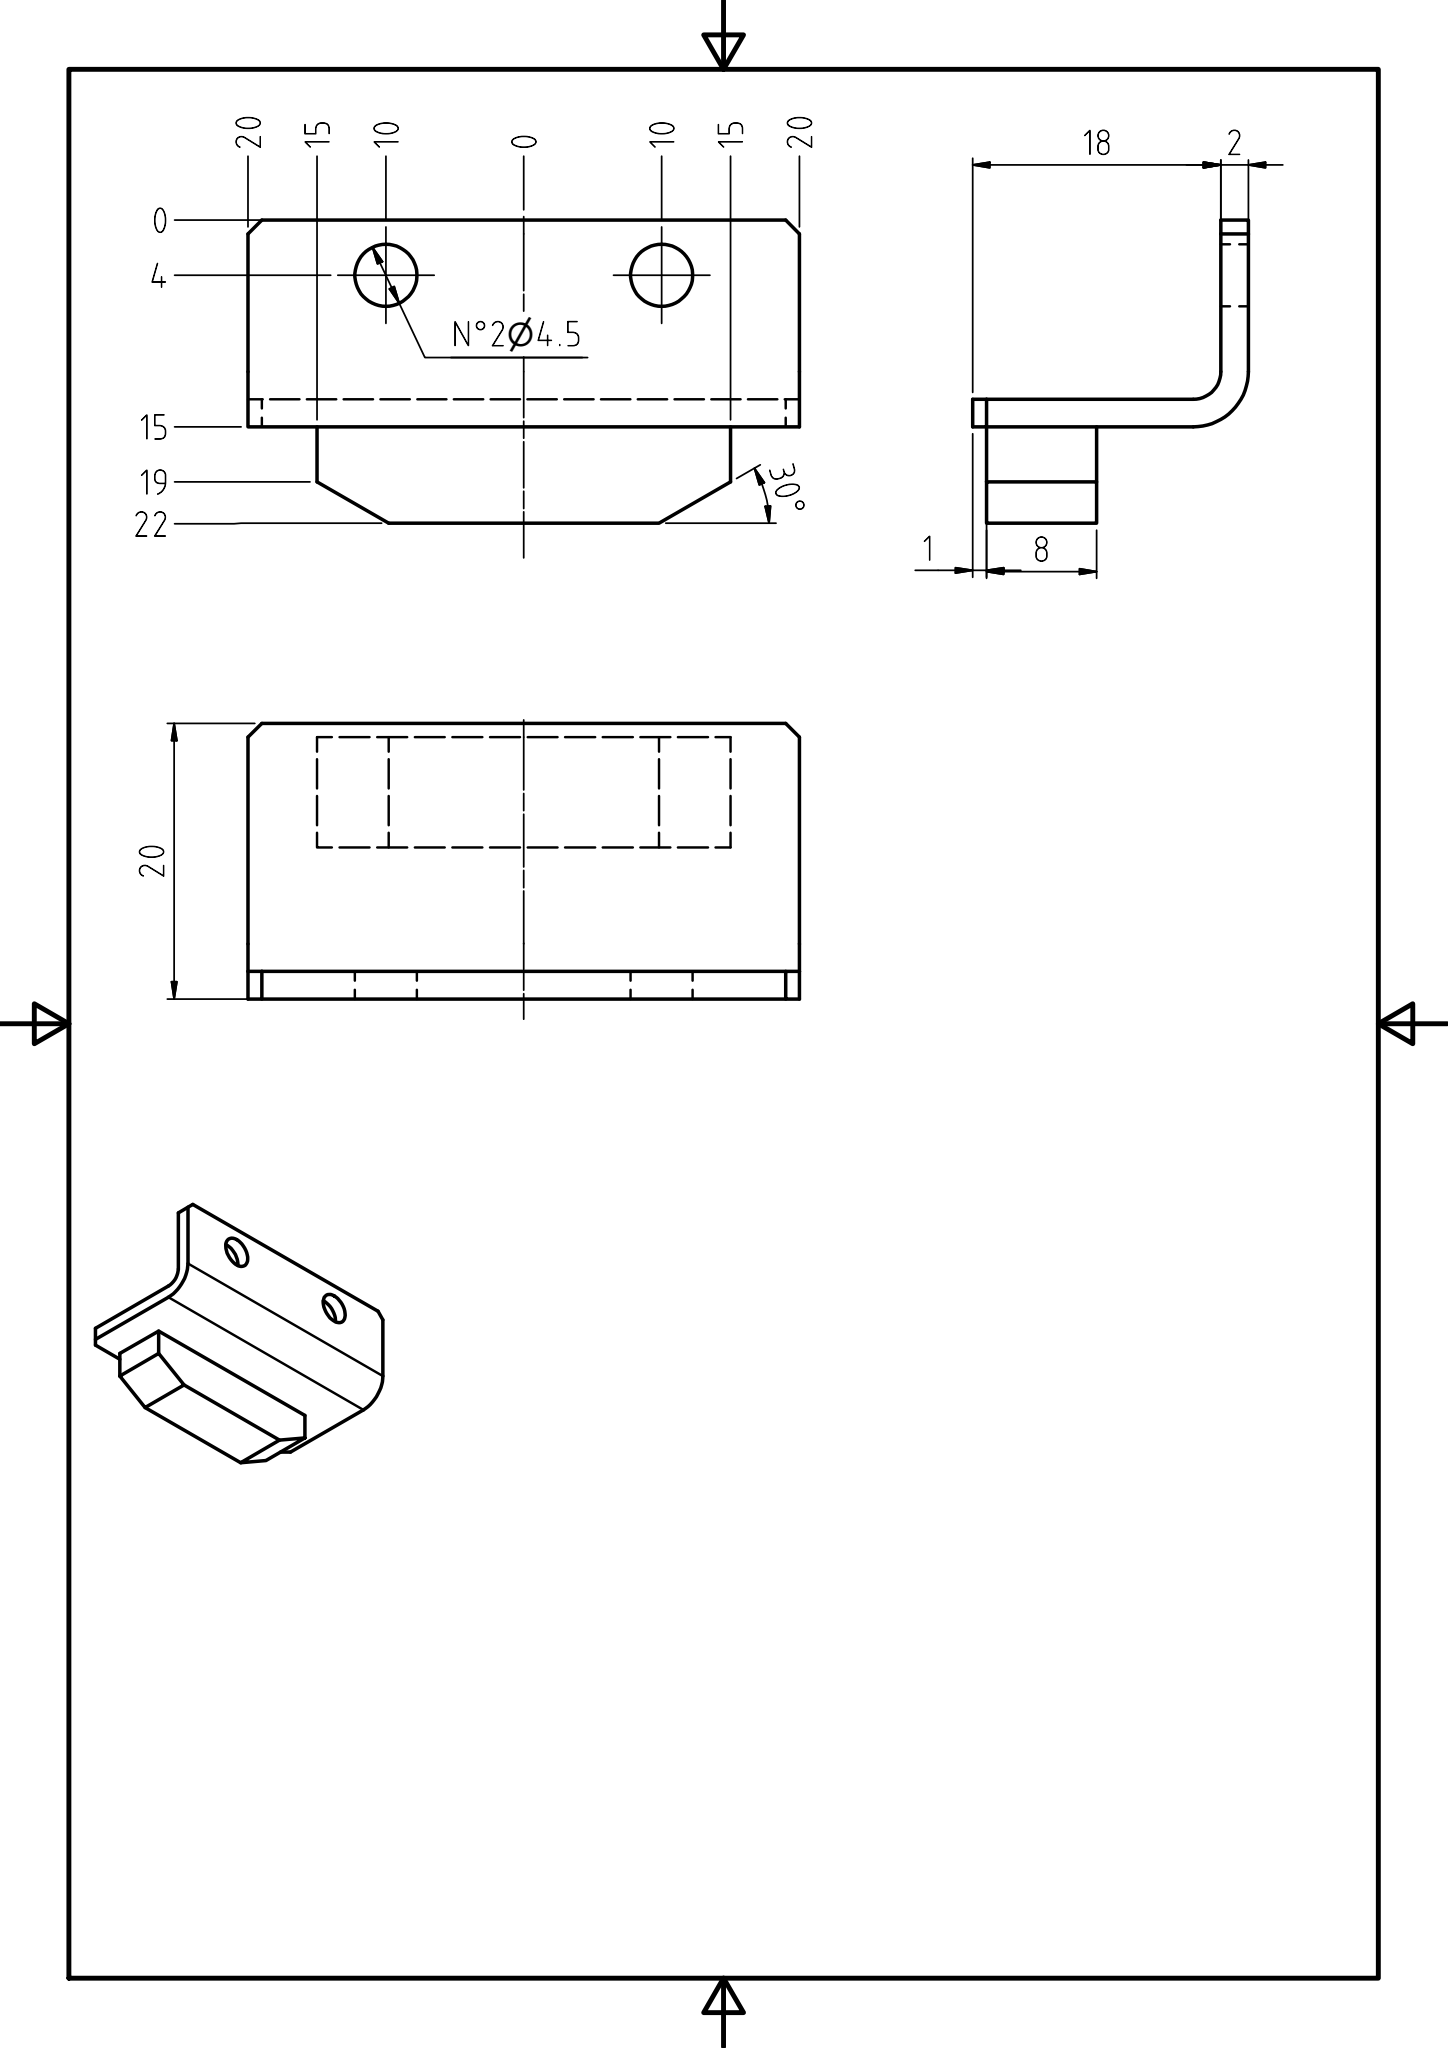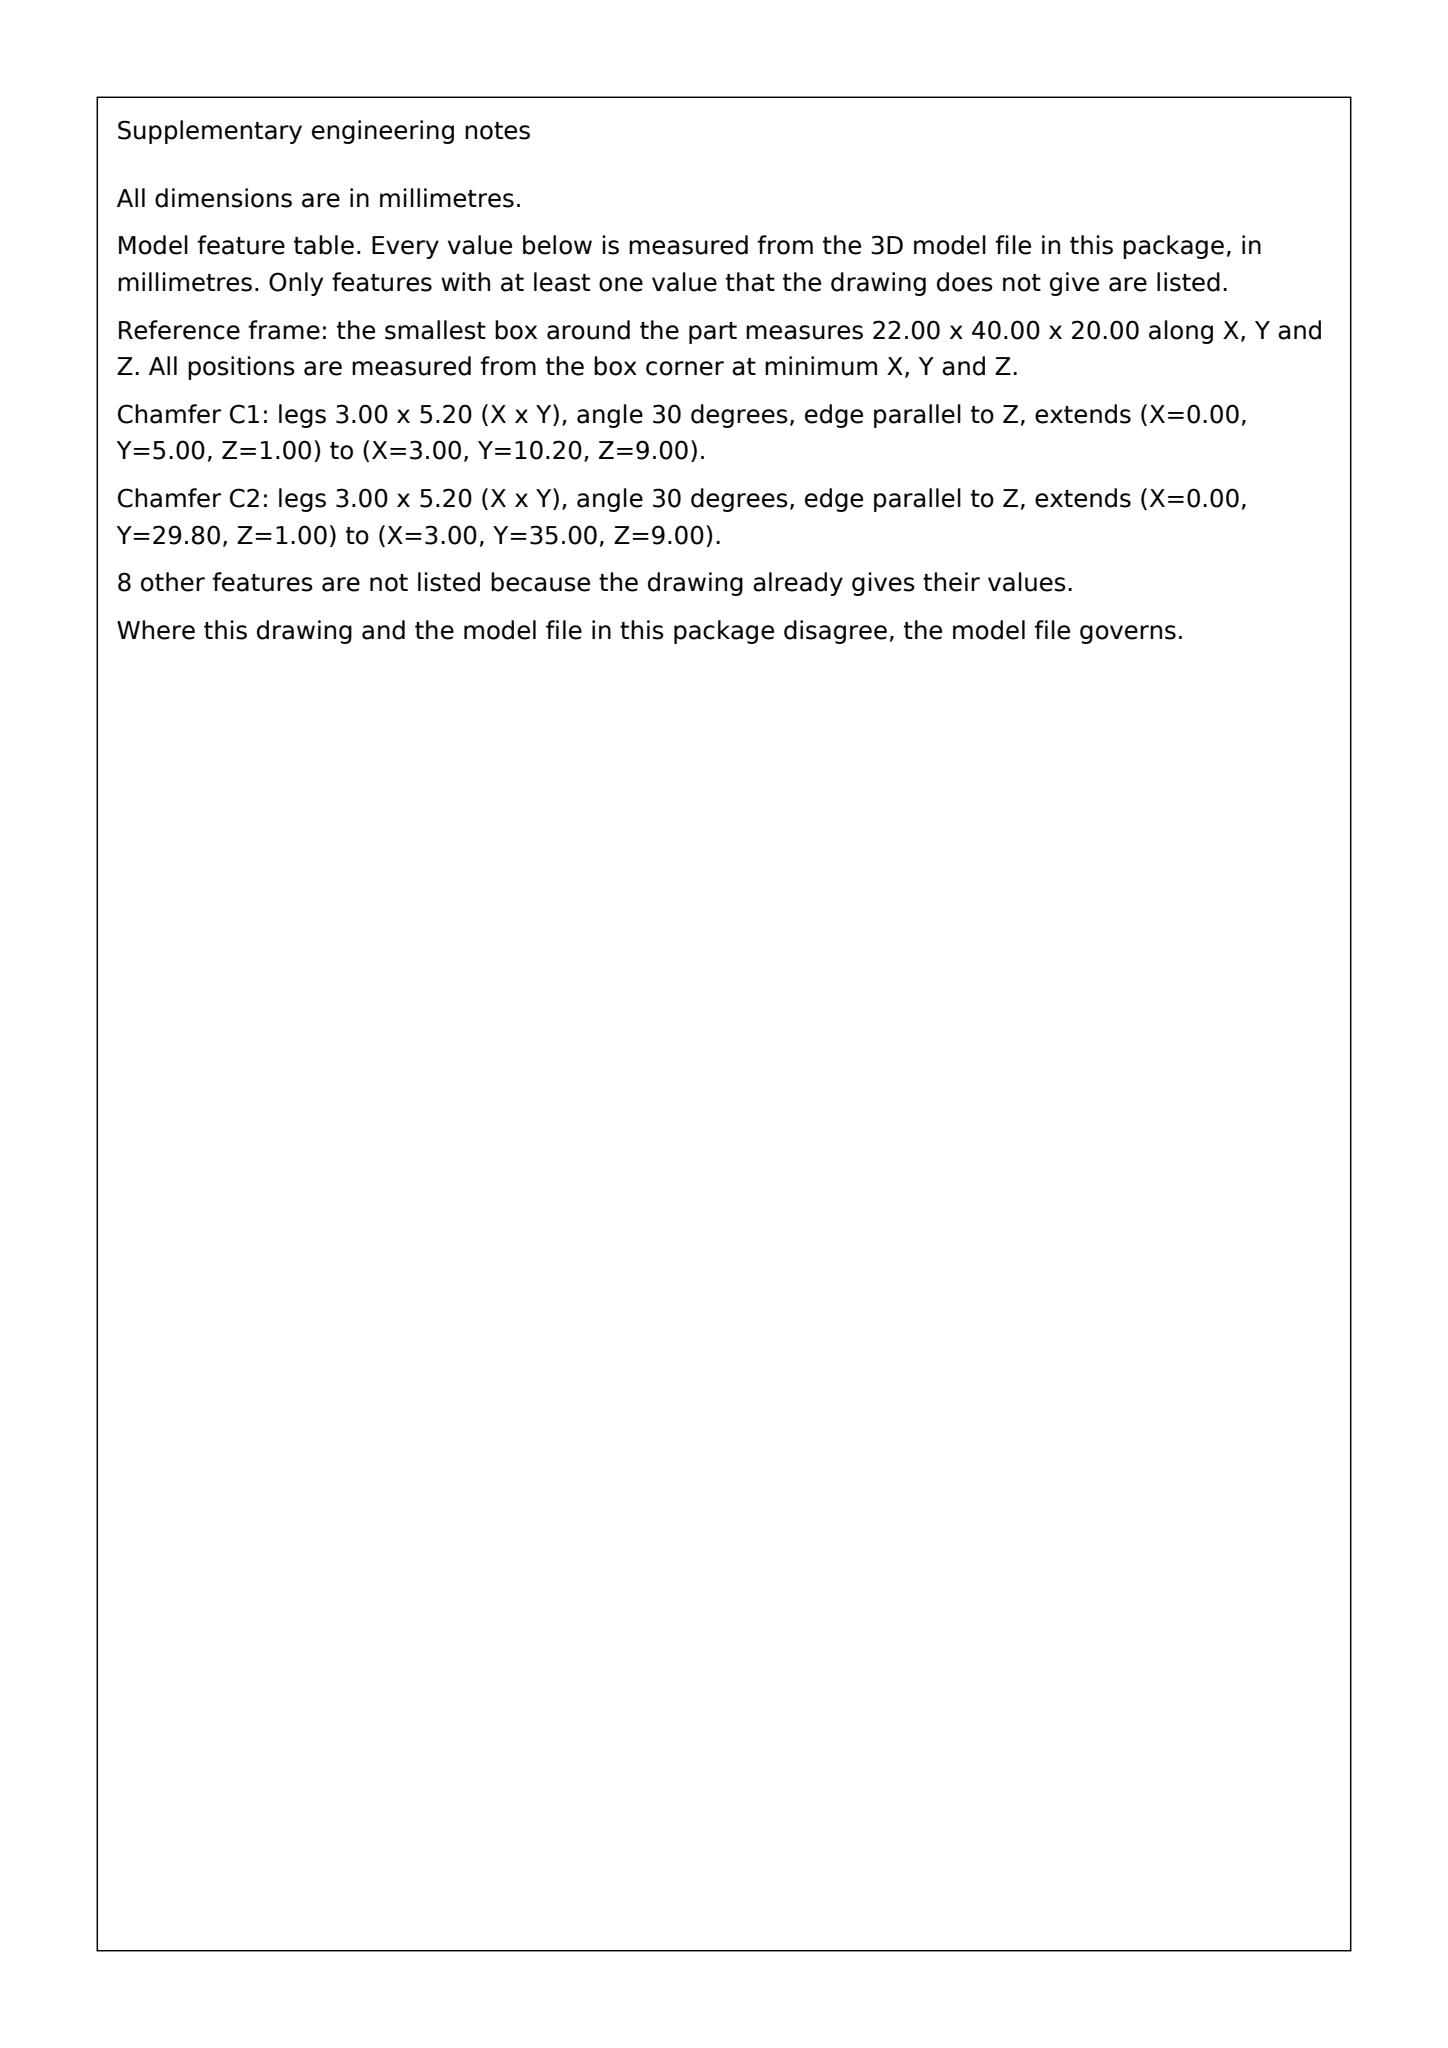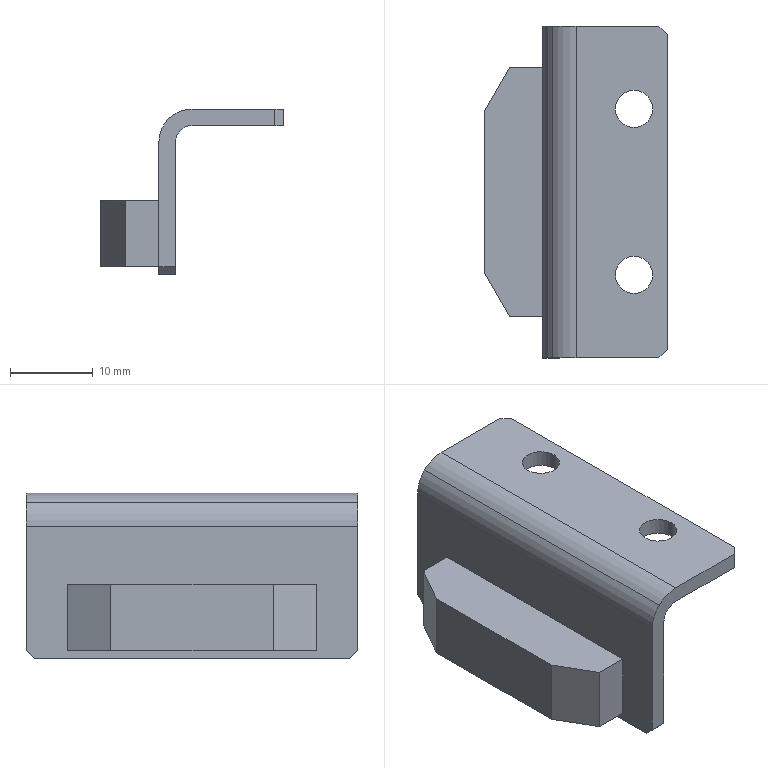Part | SolidWorks | mm | 1 solid | 27 faces | box 22 x 40 x 20 mm | volume 4025 mm3 | plane 19 | cylinder 8 | commonest cylinder face diameters 4.5 x4 4 x2 8 x2
STEP:
#1=CARTESIAN_POINT('',(-5.5,40.,6.));
#2=VERTEX_POINT('',#1);
#3=CARTESIAN_POINT('',(-4.914,40.,7.414));
#4=VERTEX_POINT('',#3);
#5=CARTESIAN_POINT('',(-3.5,40.,6.));
#6=DIRECTION('',(0.,1.,0.));
#7=DIRECTION('',(-0.7071,0.,0.7071));
#8=AXIS2_PLACEMENT_3D('',#5,#6,#7);
#9=CIRCLE('',#8,2.);
#10=EDGE_CURVE('',#2,#4,#9,.T.);
#11=ORIENTED_EDGE('',*,*,#10,.T.);
#12=CARTESIAN_POINT('',(-4.914,0.,7.414));
#13=VERTEX_POINT('',#12);
#14=CARTESIAN_POINT('',(-4.914,40.,7.414));
#15=DIRECTION('',(0.,-1.,0.));
#16=VECTOR('',#15,1000.);
#17=LINE('',#14,#16);
#18=EDGE_CURVE('',#4,#13,#17,.T.);
#19=ORIENTED_EDGE('',*,*,#18,.T.);
#20=CARTESIAN_POINT('',(-5.5,0.,6.));
#21=VERTEX_POINT('',#20);
#22=CARTESIAN_POINT('',(-3.5,0.,6.));
#23=DIRECTION('',(0.,-1.,0.));
#24=DIRECTION('',(-0.7071,0.,0.7071));
#25=AXIS2_PLACEMENT_3D('',#22,#23,#24);
#26=CIRCLE('',#25,2.);
#27=EDGE_CURVE('',#13,#21,#26,.T.);
#28=ORIENTED_EDGE('',*,*,#27,.T.);
#29=CARTESIAN_POINT('',(-5.5,40.,6.));
#30=DIRECTION('',(0.,1.,0.));
#31=VECTOR('',#30,1000.);
#32=LINE('',#29,#31);
#33=EDGE_CURVE('',#21,#2,#32,.T.);
#34=ORIENTED_EDGE('',*,*,#33,.T.);
#35=EDGE_LOOP('',(#11,#19,#28,#34));
#36=FACE_OUTER_BOUND('',#35,.T.);
#37=CARTESIAN_POINT('',(-3.5,40.,6.));
#38=DIRECTION('',(0.,-1.,0.));
#39=DIRECTION('',(-0.7071,0.,0.7071));
#40=AXIS2_PLACEMENT_3D('',#37,#38,#39);
#41=CYLINDRICAL_SURFACE('',#40,2.);
#42=ADVANCED_FACE('',(#36),#41,.F.);
#43=CARTESIAN_POINT('',(-7.5,0.,6.));
#44=VERTEX_POINT('',#43);
#45=CARTESIAN_POINT('',(-6.328,0.,8.828));
#46=VERTEX_POINT('',#45);
#47=CARTESIAN_POINT('',(-3.5,0.,6.));
#48=DIRECTION('',(0.,1.,0.));
#49=DIRECTION('',(-0.7071,0.,0.7071));
#50=AXIS2_PLACEMENT_3D('',#47,#48,#49);
#51=CIRCLE('',#50,4.);
#52=EDGE_CURVE('',#44,#46,#51,.T.);
#53=ORIENTED_EDGE('',*,*,#52,.T.);
#54=CARTESIAN_POINT('',(-6.328,40.,8.828));
#55=VERTEX_POINT('',#54);
#56=CARTESIAN_POINT('',(-6.328,0.,8.828));
#57=DIRECTION('',(0.,1.,0.));
#58=VECTOR('',#57,1000.);
#59=LINE('',#56,#58);
#60=EDGE_CURVE('',#46,#55,#59,.T.);
#61=ORIENTED_EDGE('',*,*,#60,.T.);
#62=CARTESIAN_POINT('',(-7.5,40.,6.));
#63=VERTEX_POINT('',#62);
#64=CARTESIAN_POINT('',(-3.5,40.,6.));
#65=DIRECTION('',(0.,-1.,0.));
#66=DIRECTION('',(-0.7071,0.,0.7071));
#67=AXIS2_PLACEMENT_3D('',#64,#65,#66);
#68=CIRCLE('',#67,4.);
#69=EDGE_CURVE('',#55,#63,#68,.T.);
#70=ORIENTED_EDGE('',*,*,#69,.T.);
#71=CARTESIAN_POINT('',(-7.5,0.,6.));
#72=DIRECTION('',(0.,-1.,0.));
#73=VECTOR('',#72,1000.);
#74=LINE('',#71,#73);
#75=EDGE_CURVE('',#63,#44,#74,.T.);
#76=ORIENTED_EDGE('',*,*,#75,.T.);
#77=EDGE_LOOP('',(#53,#61,#70,#76));
#78=FACE_OUTER_BOUND('',#77,.T.);
#79=CARTESIAN_POINT('',(-3.5,0.,6.));
#80=DIRECTION('',(0.,1.,0.));
#81=DIRECTION('',(-0.7071,0.,0.7071));
#82=AXIS2_PLACEMENT_3D('',#79,#80,#81);
#83=CYLINDRICAL_SURFACE('',#82,4.);
#84=ADVANCED_FACE('',(#78),#83,.T.);
#85=CARTESIAN_POINT('',(5.75,30.,10.));
#86=VERTEX_POINT('',#85);
#87=CARTESIAN_POINT('',(1.25,30.,10.));
#88=VERTEX_POINT('',#87);
#89=CARTESIAN_POINT('',(3.5,30.,10.));
#90=DIRECTION('',(-0.,0.,-1.));
#91=DIRECTION('',(-1.,0.,0.));
#92=AXIS2_PLACEMENT_3D('',#89,#90,#91);
#93=CIRCLE('',#92,2.25);
#94=EDGE_CURVE('',#86,#88,#93,.T.);
#95=ORIENTED_EDGE('',*,*,#94,.F.);
#96=CARTESIAN_POINT('',(5.75,30.,8.));
#97=VERTEX_POINT('',#96);
#98=CARTESIAN_POINT('',(5.75,30.,12.4));
#99=DIRECTION('',(-0.,0.,-1.));
#100=VECTOR('',#99,1000.);
#101=LINE('',#98,#100);
#102=EDGE_CURVE('',#86,#97,#101,.T.);
#103=ORIENTED_EDGE('',*,*,#102,.T.);
#104=CARTESIAN_POINT('',(1.25,30.,8.));
#105=VERTEX_POINT('',#104);
#106=CARTESIAN_POINT('',(3.5,30.,8.));
#107=DIRECTION('',(0.,0.,1.));
#108=DIRECTION('',(-1.,0.,0.));
#109=AXIS2_PLACEMENT_3D('',#106,#107,#108);
#110=CIRCLE('',#109,2.25);
#111=EDGE_CURVE('',#105,#97,#110,.T.);
#112=ORIENTED_EDGE('',*,*,#111,.F.);
#113=CARTESIAN_POINT('',(1.25,30.,12.4));
#114=DIRECTION('',(-0.,0.,-1.));
#115=VECTOR('',#114,1000.);
#116=LINE('',#113,#115);
#117=EDGE_CURVE('',#88,#105,#116,.T.);
#118=ORIENTED_EDGE('',*,*,#117,.F.);
#119=EDGE_LOOP('',(#95,#103,#112,#118));
#120=FACE_OUTER_BOUND('',#119,.T.);
#121=CARTESIAN_POINT('',(3.5,30.,12.4));
#122=DIRECTION('',(-0.,0.,-1.));
#123=DIRECTION('',(-1.,0.,0.));
#124=AXIS2_PLACEMENT_3D('',#121,#122,#123);
#125=CYLINDRICAL_SURFACE('',#124,2.25);
#126=ADVANCED_FACE('',(#120),#125,.F.);
#127=CARTESIAN_POINT('',(5.75,10.,10.));
#128=VERTEX_POINT('',#127);
#129=CARTESIAN_POINT('',(1.25,10.,10.));
#130=VERTEX_POINT('',#129);
#131=CARTESIAN_POINT('',(3.5,10.,10.));
#132=DIRECTION('',(-0.,0.,-1.));
#133=DIRECTION('',(-1.,0.,0.));
#134=AXIS2_PLACEMENT_3D('',#131,#132,#133);
#135=CIRCLE('',#134,2.25);
#136=EDGE_CURVE('',#128,#130,#135,.T.);
#137=ORIENTED_EDGE('',*,*,#136,.F.);
#138=CARTESIAN_POINT('',(5.75,10.,8.));
#139=VERTEX_POINT('',#138);
#140=CARTESIAN_POINT('',(5.75,10.,12.4));
#141=DIRECTION('',(-0.,0.,-1.));
#142=VECTOR('',#141,1000.);
#143=LINE('',#140,#142);
#144=EDGE_CURVE('',#128,#139,#143,.T.);
#145=ORIENTED_EDGE('',*,*,#144,.T.);
#146=CARTESIAN_POINT('',(1.25,10.,8.));
#147=VERTEX_POINT('',#146);
#148=CARTESIAN_POINT('',(3.5,10.,8.));
#149=DIRECTION('',(0.,0.,1.));
#150=DIRECTION('',(-1.,0.,0.));
#151=AXIS2_PLACEMENT_3D('',#148,#149,#150);
#152=CIRCLE('',#151,2.25);
#153=EDGE_CURVE('',#147,#139,#152,.T.);
#154=ORIENTED_EDGE('',*,*,#153,.F.);
#155=CARTESIAN_POINT('',(1.25,10.,12.4));
#156=DIRECTION('',(-0.,0.,-1.));
#157=VECTOR('',#156,1000.);
#158=LINE('',#155,#157);
#159=EDGE_CURVE('',#130,#147,#158,.T.);
#160=ORIENTED_EDGE('',*,*,#159,.F.);
#161=EDGE_LOOP('',(#137,#145,#154,#160));
#162=FACE_OUTER_BOUND('',#161,.T.);
#163=CARTESIAN_POINT('',(3.5,10.,12.4));
#164=DIRECTION('',(-0.,0.,-1.));
#165=DIRECTION('',(-1.,0.,0.));
#166=AXIS2_PLACEMENT_3D('',#163,#164,#165);
#167=CYLINDRICAL_SURFACE('',#166,2.25);
#168=ADVANCED_FACE('',(#162),#167,.F.);
#169=CARTESIAN_POINT('',(-7.5,0.,-9.));
#170=VERTEX_POINT('',#169);
#171=CARTESIAN_POINT('',(-7.5,1.,-10.));
#172=VERTEX_POINT('',#171);
#173=CARTESIAN_POINT('',(-7.5,0.5,-9.5));
#174=DIRECTION('',(0.,0.7071,-0.7071));
#175=VECTOR('',#174,1000.);
#176=LINE('',#173,#175);
#177=EDGE_CURVE('',#170,#172,#176,.T.);
#178=ORIENTED_EDGE('',*,*,#177,.T.);
#179=CARTESIAN_POINT('',(-5.5,1.,-10.));
#180=VERTEX_POINT('',#179);
#181=CARTESIAN_POINT('',(3.75,1.,-10.));
#182=DIRECTION('',(1.,0.,0.));
#183=VECTOR('',#182,1000.);
#184=LINE('',#181,#183);
#185=EDGE_CURVE('',#172,#180,#184,.T.);
#186=ORIENTED_EDGE('',*,*,#185,.T.);
#187=CARTESIAN_POINT('',(-5.5,0.,-9.));
#188=VERTEX_POINT('',#187);
#189=CARTESIAN_POINT('',(-5.5,6.,-15.));
#190=DIRECTION('',(0.,-0.7071,0.7071));
#191=VECTOR('',#190,1000.);
#192=LINE('',#189,#191);
#193=EDGE_CURVE('',#180,#188,#192,.T.);
#194=ORIENTED_EDGE('',*,*,#193,.T.);
#195=CARTESIAN_POINT('',(3.75,0.,-9.));
#196=DIRECTION('',(-1.,0.,-0.));
#197=VECTOR('',#196,1000.);
#198=LINE('',#195,#197);
#199=EDGE_CURVE('',#188,#170,#198,.T.);
#200=ORIENTED_EDGE('',*,*,#199,.T.);
#201=EDGE_LOOP('',(#178,#186,#194,#200));
#202=FACE_OUTER_BOUND('',#201,.T.);
#203=CARTESIAN_POINT('',(3.75,0.5,-9.5));
#204=DIRECTION('',(0.,-0.7071,-0.7071));
#205=DIRECTION('',(0.,-0.7071,0.7071));
#206=AXIS2_PLACEMENT_3D('',#203,#204,#205);
#207=PLANE('',#206);
#208=ADVANCED_FACE('',(#202),#207,.T.);
#209=ORIENTED_EDGE('',*,*,#199,.F.);
#210=CARTESIAN_POINT('',(-5.5,0.,4.));
#211=DIRECTION('',(0.,0.,1.));
#212=VECTOR('',#211,1000.);
#213=LINE('',#210,#212);
#214=EDGE_CURVE('',#188,#21,#213,.T.);
#215=ORIENTED_EDGE('',*,*,#214,.T.);
#216=ORIENTED_EDGE('',*,*,#27,.F.);
#217=CARTESIAN_POINT('',(-3.5,0.,8.));
#218=VERTEX_POINT('',#217);
#219=CARTESIAN_POINT('',(-3.5,0.,6.));
#220=DIRECTION('',(0.,-1.,0.));
#221=DIRECTION('',(-0.7071,0.,0.7071));
#222=AXIS2_PLACEMENT_3D('',#219,#220,#221);
#223=CIRCLE('',#222,2.);
#224=EDGE_CURVE('',#218,#13,#223,.T.);
#225=ORIENTED_EDGE('',*,*,#224,.F.);
#226=CARTESIAN_POINT('',(6.5,0.,8.));
#227=VERTEX_POINT('',#226);
#228=CARTESIAN_POINT('',(7.237,0.,8.));
#229=DIRECTION('',(1.,0.,-0.));
#230=VECTOR('',#229,1000.);
#231=LINE('',#228,#230);
#232=EDGE_CURVE('',#218,#227,#231,.T.);
#233=ORIENTED_EDGE('',*,*,#232,.T.);
#234=CARTESIAN_POINT('',(6.5,0.,10.));
#235=VERTEX_POINT('',#234);
#236=CARTESIAN_POINT('',(6.5,0.,5.));
#237=DIRECTION('',(0.,0.,-1.));
#238=VECTOR('',#237,1000.);
#239=LINE('',#236,#238);
#240=EDGE_CURVE('',#235,#227,#239,.T.);
#241=ORIENTED_EDGE('',*,*,#240,.F.);
#242=CARTESIAN_POINT('',(-3.5,0.,10.));
#243=VERTEX_POINT('',#242);
#244=CARTESIAN_POINT('',(-7.5,0.,10.));
#245=DIRECTION('',(1.,0.,-0.));
#246=VECTOR('',#245,1000.);
#247=LINE('',#244,#246);
#248=EDGE_CURVE('',#243,#235,#247,.T.);
#249=ORIENTED_EDGE('',*,*,#248,.F.);
#250=CARTESIAN_POINT('',(-3.5,0.,6.));
#251=DIRECTION('',(0.,1.,0.));
#252=DIRECTION('',(-0.7071,0.,0.7071));
#253=AXIS2_PLACEMENT_3D('',#250,#251,#252);
#254=CIRCLE('',#253,4.);
#255=EDGE_CURVE('',#46,#243,#254,.T.);
#256=ORIENTED_EDGE('',*,*,#255,.F.);
#257=ORIENTED_EDGE('',*,*,#52,.F.);
#258=CARTESIAN_POINT('',(-7.5,0.,-10.));
#259=DIRECTION('',(0.,0.,1.));
#260=VECTOR('',#259,1000.);
#261=LINE('',#258,#260);
#262=EDGE_CURVE('',#170,#44,#261,.T.);
#263=ORIENTED_EDGE('',*,*,#262,.F.);
#264=EDGE_LOOP('',(#209,#215,#216,#225,#233,#241,#249,#256,#257,#263));
#265=FACE_OUTER_BOUND('',#264,.T.);
#266=CARTESIAN_POINT('',(0.,0.,0.));
#267=DIRECTION('',(0.,1.,0.));
#268=DIRECTION('',(1.,0.,0.));
#269=AXIS2_PLACEMENT_3D('',#266,#267,#268);
#270=PLANE('',#269);
#271=ADVANCED_FACE('',(#265),#270,.F.);
#272=ORIENTED_EDGE('',*,*,#193,.F.);
#273=CARTESIAN_POINT('',(-5.5,39.,-10.));
#274=VERTEX_POINT('',#273);
#275=CARTESIAN_POINT('',(-5.5,20.,-10.));
#276=DIRECTION('',(0.,-1.,0.));
#277=VECTOR('',#276,1000.);
#278=LINE('',#275,#277);
#279=EDGE_CURVE('',#274,#180,#278,.T.);
#280=ORIENTED_EDGE('',*,*,#279,.F.);
#281=CARTESIAN_POINT('',(-5.5,40.,-9.));
#282=VERTEX_POINT('',#281);
#283=CARTESIAN_POINT('',(-5.5,44.,-5.));
#284=DIRECTION('',(-0.,-0.7071,-0.7071));
#285=VECTOR('',#284,1000.);
#286=LINE('',#283,#285);
#287=EDGE_CURVE('',#282,#274,#286,.T.);
#288=ORIENTED_EDGE('',*,*,#287,.F.);
#289=CARTESIAN_POINT('',(-5.5,40.,4.));
#290=DIRECTION('',(-0.,0.,-1.));
#291=VECTOR('',#290,1000.);
#292=LINE('',#289,#291);
#293=EDGE_CURVE('',#2,#282,#292,.T.);
#294=ORIENTED_EDGE('',*,*,#293,.F.);
#295=ORIENTED_EDGE('',*,*,#33,.F.);
#296=ORIENTED_EDGE('',*,*,#214,.F.);
#297=EDGE_LOOP('',(#272,#280,#288,#294,#295,#296));
#298=FACE_OUTER_BOUND('',#297,.T.);
#299=CARTESIAN_POINT('',(-5.5,40.,8.));
#300=DIRECTION('',(-1.,0.,0.));
#301=DIRECTION('',(0.,1.,0.));
#302=AXIS2_PLACEMENT_3D('',#299,#300,#301);
#303=PLANE('',#302);
#304=ADVANCED_FACE('',(#298),#303,.F.);
#305=CARTESIAN_POINT('',(-7.5,39.,-10.));
#306=VERTEX_POINT('',#305);
#307=CARTESIAN_POINT('',(-7.5,40.,-9.));
#308=VERTEX_POINT('',#307);
#309=CARTESIAN_POINT('',(-7.5,29.5,-19.5));
#310=DIRECTION('',(0.,0.7071,0.7071));
#311=VECTOR('',#310,1000.);
#312=LINE('',#309,#311);
#313=EDGE_CURVE('',#306,#308,#312,.T.);
#314=ORIENTED_EDGE('',*,*,#313,.T.);
#315=CARTESIAN_POINT('',(3.75,40.,-9.));
#316=DIRECTION('',(1.,0.,0.));
#317=VECTOR('',#316,1000.);
#318=LINE('',#315,#317);
#319=EDGE_CURVE('',#308,#282,#318,.T.);
#320=ORIENTED_EDGE('',*,*,#319,.T.);
#321=ORIENTED_EDGE('',*,*,#287,.T.);
#322=CARTESIAN_POINT('',(3.75,39.,-10.));
#323=DIRECTION('',(-1.,0.,-0.));
#324=VECTOR('',#323,1000.);
#325=LINE('',#322,#324);
#326=EDGE_CURVE('',#274,#306,#325,.T.);
#327=ORIENTED_EDGE('',*,*,#326,.T.);
#328=EDGE_LOOP('',(#314,#320,#321,#327));
#329=FACE_OUTER_BOUND('',#328,.T.);
#330=CARTESIAN_POINT('',(3.75,39.5,-9.5));
#331=DIRECTION('',(0.,0.7071,-0.7071));
#332=DIRECTION('',(-1.,0.,-0.));
#333=AXIS2_PLACEMENT_3D('',#330,#331,#332);
#334=PLANE('',#333);
#335=ADVANCED_FACE('',(#329),#334,.T.);
#336=ORIENTED_EDGE('',*,*,#319,.F.);
#337=CARTESIAN_POINT('',(-7.5,40.,-10.));
#338=DIRECTION('',(0.,0.,1.));
#339=VECTOR('',#338,1000.);
#340=LINE('',#337,#339);
#341=EDGE_CURVE('',#308,#63,#340,.T.);
#342=ORIENTED_EDGE('',*,*,#341,.T.);
#343=ORIENTED_EDGE('',*,*,#69,.F.);
#344=CARTESIAN_POINT('',(-3.5,40.,10.));
#345=VERTEX_POINT('',#344);
#346=CARTESIAN_POINT('',(-3.5,40.,6.));
#347=DIRECTION('',(0.,-1.,0.));
#348=DIRECTION('',(-0.7071,0.,0.7071));
#349=AXIS2_PLACEMENT_3D('',#346,#347,#348);
#350=CIRCLE('',#349,4.);
#351=EDGE_CURVE('',#345,#55,#350,.T.);
#352=ORIENTED_EDGE('',*,*,#351,.F.);
#353=CARTESIAN_POINT('',(6.5,40.,10.));
#354=VERTEX_POINT('',#353);
#355=CARTESIAN_POINT('',(-7.5,40.,10.));
#356=DIRECTION('',(1.,0.,-0.));
#357=VECTOR('',#356,1000.);
#358=LINE('',#355,#357);
#359=EDGE_CURVE('',#345,#354,#358,.T.);
#360=ORIENTED_EDGE('',*,*,#359,.T.);
#361=CARTESIAN_POINT('',(6.5,40.,8.));
#362=VERTEX_POINT('',#361);
#363=CARTESIAN_POINT('',(6.5,40.,5.));
#364=DIRECTION('',(0.,0.,1.));
#365=VECTOR('',#364,1000.);
#366=LINE('',#363,#365);
#367=EDGE_CURVE('',#362,#354,#366,.T.);
#368=ORIENTED_EDGE('',*,*,#367,.F.);
#369=CARTESIAN_POINT('',(-3.5,40.,8.));
#370=VERTEX_POINT('',#369);
#371=CARTESIAN_POINT('',(7.237,40.,8.));
#372=DIRECTION('',(-1.,0.,0.));
#373=VECTOR('',#372,1000.);
#374=LINE('',#371,#373);
#375=EDGE_CURVE('',#362,#370,#374,.T.);
#376=ORIENTED_EDGE('',*,*,#375,.T.);
#377=CARTESIAN_POINT('',(-3.5,40.,6.));
#378=DIRECTION('',(0.,1.,0.));
#379=DIRECTION('',(-0.7071,0.,0.7071));
#380=AXIS2_PLACEMENT_3D('',#377,#378,#379);
#381=CIRCLE('',#380,2.);
#382=EDGE_CURVE('',#4,#370,#381,.T.);
#383=ORIENTED_EDGE('',*,*,#382,.F.);
#384=ORIENTED_EDGE('',*,*,#10,.F.);
#385=ORIENTED_EDGE('',*,*,#293,.T.);
#386=EDGE_LOOP('',(#336,#342,#343,#352,#360,#368,#376,#383,#384,#385));
#387=FACE_OUTER_BOUND('',#386,.T.);
#388=CARTESIAN_POINT('',(0.,40.,0.));
#389=DIRECTION('',(0.,1.,0.));
#390=DIRECTION('',(1.,0.,0.));
#391=AXIS2_PLACEMENT_3D('',#388,#389,#390);
#392=PLANE('',#391);
#393=ADVANCED_FACE('',(#387),#392,.T.);
#394=CARTESIAN_POINT('',(7.5,39.,8.));
#395=VERTEX_POINT('',#394);
#396=CARTESIAN_POINT('',(8.744,37.756,8.));
#397=DIRECTION('',(-0.7071,0.7071,0.));
#398=VECTOR('',#397,1000.);
#399=LINE('',#396,#398);
#400=EDGE_CURVE('',#395,#362,#399,.T.);
#401=ORIENTED_EDGE('',*,*,#400,.T.);
#402=ORIENTED_EDGE('',*,*,#367,.T.);
#403=CARTESIAN_POINT('',(7.5,39.,10.));
#404=VERTEX_POINT('',#403);
#405=CARTESIAN_POINT('',(13.25,33.25,10.));
#406=DIRECTION('',(0.7071,-0.7071,-0.));
#407=VECTOR('',#406,1000.);
#408=LINE('',#405,#407);
#409=EDGE_CURVE('',#354,#404,#408,.T.);
#410=ORIENTED_EDGE('',*,*,#409,.T.);
#411=CARTESIAN_POINT('',(7.5,39.,5.));
#412=DIRECTION('',(0.,0.,-1.));
#413=VECTOR('',#412,1000.);
#414=LINE('',#411,#413);
#415=EDGE_CURVE('',#404,#395,#414,.T.);
#416=ORIENTED_EDGE('',*,*,#415,.T.);
#417=EDGE_LOOP('',(#401,#402,#410,#416));
#418=FACE_OUTER_BOUND('',#417,.T.);
#419=CARTESIAN_POINT('',(7.,39.5,5.));
#420=DIRECTION('',(0.7071,0.7071,0.));
#421=DIRECTION('',(0.,0.,-1.));
#422=AXIS2_PLACEMENT_3D('',#419,#420,#421);
#423=PLANE('',#422);
#424=ADVANCED_FACE('',(#418),#423,.T.);
#425=ORIENTED_EDGE('',*,*,#400,.F.);
#426=CARTESIAN_POINT('',(7.5,1.,8.));
#427=VERTEX_POINT('',#426);
#428=CARTESIAN_POINT('',(7.5,20.,8.));
#429=DIRECTION('',(0.,1.,0.));
#430=VECTOR('',#429,1000.);
#431=LINE('',#428,#430);
#432=EDGE_CURVE('',#427,#395,#431,.T.);
#433=ORIENTED_EDGE('',*,*,#432,.F.);
#434=CARTESIAN_POINT('',(18.744,12.244,8.));
#435=DIRECTION('',(0.7071,0.7071,-0.));
#436=VECTOR('',#435,1000.);
#437=LINE('',#434,#436);
#438=EDGE_CURVE('',#227,#427,#437,.T.);
#439=ORIENTED_EDGE('',*,*,#438,.F.);
#440=ORIENTED_EDGE('',*,*,#232,.F.);
#441=CARTESIAN_POINT('',(-3.5,40.,8.));
#442=DIRECTION('',(0.,-1.,0.));
#443=VECTOR('',#442,1000.);
#444=LINE('',#441,#443);
#445=EDGE_CURVE('',#370,#218,#444,.T.);
#446=ORIENTED_EDGE('',*,*,#445,.F.);
#447=ORIENTED_EDGE('',*,*,#375,.F.);
#448=EDGE_LOOP('',(#425,#433,#439,#440,#446,#447));
#449=FACE_OUTER_BOUND('',#448,.T.);
#450=ORIENTED_EDGE('',*,*,#111,.T.);
#451=CARTESIAN_POINT('',(3.5,30.,8.));
#452=DIRECTION('',(0.,0.,1.));
#453=DIRECTION('',(-1.,0.,0.));
#454=AXIS2_PLACEMENT_3D('',#451,#452,#453);
#455=CIRCLE('',#454,2.25);
#456=EDGE_CURVE('',#97,#105,#455,.T.);
#457=ORIENTED_EDGE('',*,*,#456,.T.);
#458=EDGE_LOOP('',(#450,#457));
#459=FACE_BOUND('',#458,.T.);
#460=ORIENTED_EDGE('',*,*,#153,.T.);
#461=CARTESIAN_POINT('',(3.5,10.,8.));
#462=DIRECTION('',(0.,0.,1.));
#463=DIRECTION('',(-1.,0.,0.));
#464=AXIS2_PLACEMENT_3D('',#461,#462,#463);
#465=CIRCLE('',#464,2.25);
#466=EDGE_CURVE('',#139,#147,#465,.T.);
#467=ORIENTED_EDGE('',*,*,#466,.T.);
#468=EDGE_LOOP('',(#460,#467));
#469=FACE_BOUND('',#468,.T.);
#470=CARTESIAN_POINT('',(14.474,40.,8.));
#471=DIRECTION('',(0.,0.,1.));
#472=DIRECTION('',(1.,-0.,0.));
#473=AXIS2_PLACEMENT_3D('',#470,#471,#472);
#474=PLANE('',#473);
#475=ADVANCED_FACE('',(#449,#459,#469),#474,.F.);
#476=ORIENTED_EDGE('',*,*,#438,.T.);
#477=CARTESIAN_POINT('',(7.5,1.,10.));
#478=VERTEX_POINT('',#477);
#479=CARTESIAN_POINT('',(7.5,1.,5.));
#480=DIRECTION('',(0.,0.,1.));
#481=VECTOR('',#480,1000.);
#482=LINE('',#479,#481);
#483=EDGE_CURVE('',#427,#478,#482,.T.);
#484=ORIENTED_EDGE('',*,*,#483,.T.);
#485=CARTESIAN_POINT('',(3.25,-3.25,10.));
#486=DIRECTION('',(-0.7071,-0.7071,0.));
#487=VECTOR('',#486,1000.);
#488=LINE('',#485,#487);
#489=EDGE_CURVE('',#478,#235,#488,.T.);
#490=ORIENTED_EDGE('',*,*,#489,.T.);
#491=ORIENTED_EDGE('',*,*,#240,.T.);
#492=EDGE_LOOP('',(#476,#484,#490,#491));
#493=FACE_OUTER_BOUND('',#492,.T.);
#494=CARTESIAN_POINT('',(7.,0.5,5.));
#495=DIRECTION('',(0.7071,-0.7071,0.));
#496=DIRECTION('',(0.,0.,-1.));
#497=AXIS2_PLACEMENT_3D('',#494,#495,#496);
#498=PLANE('',#497);
#499=ADVANCED_FACE('',(#493),#498,.T.);
#500=ORIENTED_EDGE('',*,*,#409,.F.);
#501=ORIENTED_EDGE('',*,*,#359,.F.);
#502=CARTESIAN_POINT('',(-3.5,0.,10.));
#503=DIRECTION('',(0.,1.,0.));
#504=VECTOR('',#503,1000.);
#505=LINE('',#502,#504);
#506=EDGE_CURVE('',#243,#345,#505,.T.);
#507=ORIENTED_EDGE('',*,*,#506,.F.);
#508=ORIENTED_EDGE('',*,*,#248,.T.);
#509=ORIENTED_EDGE('',*,*,#489,.F.);
#510=CARTESIAN_POINT('',(7.5,0.,10.));
#511=DIRECTION('',(0.,1.,0.));
#512=VECTOR('',#511,1000.);
#513=LINE('',#510,#512);
#514=EDGE_CURVE('',#478,#404,#513,.T.);
#515=ORIENTED_EDGE('',*,*,#514,.T.);
#516=EDGE_LOOP('',(#500,#501,#507,#508,#509,#515));
#517=FACE_OUTER_BOUND('',#516,.T.);
#518=CARTESIAN_POINT('',(3.5,30.,10.));
#519=DIRECTION('',(-0.,0.,-1.));
#520=DIRECTION('',(-1.,0.,0.));
#521=AXIS2_PLACEMENT_3D('',#518,#519,#520);
#522=CIRCLE('',#521,2.25);
#523=EDGE_CURVE('',#88,#86,#522,.T.);
#524=ORIENTED_EDGE('',*,*,#523,.T.);
#525=ORIENTED_EDGE('',*,*,#94,.T.);
#526=EDGE_LOOP('',(#524,#525));
#527=FACE_BOUND('',#526,.T.);
#528=CARTESIAN_POINT('',(3.5,10.,10.));
#529=DIRECTION('',(-0.,0.,-1.));
#530=DIRECTION('',(-1.,0.,0.));
#531=AXIS2_PLACEMENT_3D('',#528,#529,#530);
#532=CIRCLE('',#531,2.25);
#533=EDGE_CURVE('',#130,#128,#532,.T.);
#534=ORIENTED_EDGE('',*,*,#533,.T.);
#535=ORIENTED_EDGE('',*,*,#136,.T.);
#536=EDGE_LOOP('',(#534,#535));
#537=FACE_BOUND('',#536,.T.);
#538=CARTESIAN_POINT('',(-7.5,0.,10.));
#539=DIRECTION('',(0.,0.,1.));
#540=DIRECTION('',(1.,-0.,0.));
#541=AXIS2_PLACEMENT_3D('',#538,#539,#540);
#542=PLANE('',#541);
#543=ADVANCED_FACE('',(#517,#527,#537),#542,.T.);
#544=ORIENTED_EDGE('',*,*,#144,.F.);
#545=ORIENTED_EDGE('',*,*,#533,.F.);
#546=ORIENTED_EDGE('',*,*,#159,.T.);
#547=ORIENTED_EDGE('',*,*,#466,.F.);
#548=EDGE_LOOP('',(#544,#545,#546,#547));
#549=FACE_OUTER_BOUND('',#548,.T.);
#550=CARTESIAN_POINT('',(3.5,10.,12.4));
#551=DIRECTION('',(-0.,0.,-1.));
#552=DIRECTION('',(-1.,0.,0.));
#553=AXIS2_PLACEMENT_3D('',#550,#551,#552);
#554=CYLINDRICAL_SURFACE('',#553,2.25);
#555=ADVANCED_FACE('',(#549),#554,.F.);
#556=ORIENTED_EDGE('',*,*,#102,.F.);
#557=ORIENTED_EDGE('',*,*,#523,.F.);
#558=ORIENTED_EDGE('',*,*,#117,.T.);
#559=ORIENTED_EDGE('',*,*,#456,.F.);
#560=EDGE_LOOP('',(#556,#557,#558,#559));
#561=FACE_OUTER_BOUND('',#560,.T.);
#562=CARTESIAN_POINT('',(3.5,30.,12.4));
#563=DIRECTION('',(-0.,0.,-1.));
#564=DIRECTION('',(-1.,0.,0.));
#565=AXIS2_PLACEMENT_3D('',#562,#563,#564);
#566=CYLINDRICAL_SURFACE('',#565,2.25);
#567=ADVANCED_FACE('',(#561),#566,.F.);
#568=CARTESIAN_POINT('',(-11.5,5.,-1.));
#569=VERTEX_POINT('',#568);
#570=CARTESIAN_POINT('',(-14.5,10.196,-1.));
#571=VERTEX_POINT('',#570);
#572=CARTESIAN_POINT('',(-11.75,5.433,-1.));
#573=DIRECTION('',(-0.5,0.866,-0.));
#574=VECTOR('',#573,1000.);
#575=LINE('',#572,#574);
#576=EDGE_CURVE('',#569,#571,#575,.T.);
#577=ORIENTED_EDGE('',*,*,#576,.T.);
#578=CARTESIAN_POINT('',(-14.5,10.196,-9.));
#579=VERTEX_POINT('',#578);
#580=CARTESIAN_POINT('',(-14.5,10.196,-7.));
#581=DIRECTION('',(0.,0.,-1.));
#582=VECTOR('',#581,1000.);
#583=LINE('',#580,#582);
#584=EDGE_CURVE('',#571,#579,#583,.T.);
#585=ORIENTED_EDGE('',*,*,#584,.T.);
#586=CARTESIAN_POINT('',(-11.5,5.,-9.));
#587=VERTEX_POINT('',#586);
#588=CARTESIAN_POINT('',(-18.245,16.683,-9.));
#589=DIRECTION('',(0.5,-0.866,0.));
#590=VECTOR('',#589,1000.);
#591=LINE('',#588,#590);
#592=EDGE_CURVE('',#579,#587,#591,.T.);
#593=ORIENTED_EDGE('',*,*,#592,.T.);
#594=CARTESIAN_POINT('',(-11.5,5.,-7.));
#595=DIRECTION('',(0.,0.,1.));
#596=VECTOR('',#595,1000.);
#597=LINE('',#594,#596);
#598=EDGE_CURVE('',#587,#569,#597,.T.);
#599=ORIENTED_EDGE('',*,*,#598,.T.);
#600=EDGE_LOOP('',(#577,#585,#593,#599));
#601=FACE_OUTER_BOUND('',#600,.T.);
#602=CARTESIAN_POINT('',(-13.,7.598,-7.));
#603=DIRECTION('',(-0.866,-0.5,0.));
#604=DIRECTION('',(-0.5,0.866,0.));
#605=AXIS2_PLACEMENT_3D('',#602,#603,#604);
#606=PLANE('',#605);
#607=ADVANCED_FACE('',(#601),#606,.T.);
#608=ORIENTED_EDGE('',*,*,#592,.F.);
#609=CARTESIAN_POINT('',(-14.5,29.804,-9.));
#610=VERTEX_POINT('',#609);
#611=CARTESIAN_POINT('',(-14.5,35.,-9.));
#612=DIRECTION('',(0.,-1.,0.));
#613=VECTOR('',#612,1000.);
#614=LINE('',#611,#613);
#615=EDGE_CURVE('',#610,#579,#614,.T.);
#616=ORIENTED_EDGE('',*,*,#615,.F.);
#617=CARTESIAN_POINT('',(-11.5,35.,-9.));
#618=VERTEX_POINT('',#617);
#619=CARTESIAN_POINT('',(-11.75,34.567,-9.));
#620=DIRECTION('',(-0.5,-0.866,0.));
#621=VECTOR('',#620,1000.);
#622=LINE('',#619,#621);
#623=EDGE_CURVE('',#618,#610,#622,.T.);
#624=ORIENTED_EDGE('',*,*,#623,.F.);
#625=CARTESIAN_POINT('',(-7.5,35.,-9.));
#626=VERTEX_POINT('',#625);
#627=CARTESIAN_POINT('',(-7.5,35.,-9.));
#628=DIRECTION('',(-1.,0.,0.));
#629=VECTOR('',#628,1000.);
#630=LINE('',#627,#629);
#631=EDGE_CURVE('',#626,#618,#630,.T.);
#632=ORIENTED_EDGE('',*,*,#631,.F.);
#633=CARTESIAN_POINT('',(-7.5,5.,-9.));
#634=VERTEX_POINT('',#633);
#635=CARTESIAN_POINT('',(-7.5,17.5,-9.));
#636=DIRECTION('',(0.,1.,-0.));
#637=VECTOR('',#636,1000.);
#638=LINE('',#635,#637);
#639=EDGE_CURVE('',#634,#626,#638,.T.);
#640=ORIENTED_EDGE('',*,*,#639,.F.);
#641=CARTESIAN_POINT('',(-7.5,5.,-9.));
#642=DIRECTION('',(-1.,0.,0.));
#643=VECTOR('',#642,1000.);
#644=LINE('',#641,#643);
#645=EDGE_CURVE('',#634,#587,#644,.T.);
#646=ORIENTED_EDGE('',*,*,#645,.T.);
#647=EDGE_LOOP('',(#608,#616,#624,#632,#640,#646));
#648=FACE_OUTER_BOUND('',#647,.T.);
#649=CARTESIAN_POINT('',(-7.5,35.,-9.));
#650=DIRECTION('',(0.,-0.,-1.));
#651=DIRECTION('',(0.,-1.,0.));
#652=AXIS2_PLACEMENT_3D('',#649,#650,#651);
#653=PLANE('',#652);
#654=ADVANCED_FACE('',(#648),#653,.T.);
#655=ORIENTED_EDGE('',*,*,#584,.F.);
#656=CARTESIAN_POINT('',(-14.5,29.804,-1.));
#657=VERTEX_POINT('',#656);
#658=CARTESIAN_POINT('',(-14.5,5.,-1.));
#659=DIRECTION('',(0.,1.,-0.));
#660=VECTOR('',#659,1000.);
#661=LINE('',#658,#660);
#662=EDGE_CURVE('',#571,#657,#661,.T.);
#663=ORIENTED_EDGE('',*,*,#662,.T.);
#664=CARTESIAN_POINT('',(-14.5,29.804,-3.));
#665=DIRECTION('',(0.,0.,1.));
#666=VECTOR('',#665,1000.);
#667=LINE('',#664,#666);
#668=EDGE_CURVE('',#610,#657,#667,.T.);
#669=ORIENTED_EDGE('',*,*,#668,.F.);
#670=ORIENTED_EDGE('',*,*,#615,.T.);
#671=EDGE_LOOP('',(#655,#663,#669,#670));
#672=FACE_OUTER_BOUND('',#671,.T.);
#673=CARTESIAN_POINT('',(-14.5,20.,-5.));
#674=DIRECTION('',(-1.,0.,0.));
#675=DIRECTION('',(0.,0.,1.));
#676=AXIS2_PLACEMENT_3D('',#673,#674,#675);
#677=PLANE('',#676);
#678=ADVANCED_FACE('',(#672),#677,.T.);
#679=ORIENTED_EDGE('',*,*,#623,.T.);
#680=ORIENTED_EDGE('',*,*,#668,.T.);
#681=CARTESIAN_POINT('',(-11.5,35.,-1.));
#682=VERTEX_POINT('',#681);
#683=CARTESIAN_POINT('',(-18.245,23.317,-1.));
#684=DIRECTION('',(0.5,0.866,-0.));
#685=VECTOR('',#684,1000.);
#686=LINE('',#683,#685);
#687=EDGE_CURVE('',#657,#682,#686,.T.);
#688=ORIENTED_EDGE('',*,*,#687,.T.);
#689=CARTESIAN_POINT('',(-11.5,35.,-3.));
#690=DIRECTION('',(0.,0.,-1.));
#691=VECTOR('',#690,1000.);
#692=LINE('',#689,#691);
#693=EDGE_CURVE('',#682,#618,#692,.T.);
#694=ORIENTED_EDGE('',*,*,#693,.T.);
#695=EDGE_LOOP('',(#679,#680,#688,#694));
#696=FACE_OUTER_BOUND('',#695,.T.);
#697=CARTESIAN_POINT('',(-13.,32.402,-3.));
#698=DIRECTION('',(-0.866,0.5,0.));
#699=DIRECTION('',(0.,0.,1.));
#700=AXIS2_PLACEMENT_3D('',#697,#698,#699);
#701=PLANE('',#700);
#702=ADVANCED_FACE('',(#696),#701,.T.);
#703=ORIENTED_EDGE('',*,*,#598,.F.);
#704=ORIENTED_EDGE('',*,*,#645,.F.);
#705=CARTESIAN_POINT('',(-7.5,5.,-1.));
#706=VERTEX_POINT('',#705);
#707=CARTESIAN_POINT('',(-7.5,5.,-9.5));
#708=DIRECTION('',(0.,0.,-1.));
#709=VECTOR('',#708,1000.);
#710=LINE('',#707,#709);
#711=EDGE_CURVE('',#706,#634,#710,.T.);
#712=ORIENTED_EDGE('',*,*,#711,.F.);
#713=CARTESIAN_POINT('',(-7.5,5.,-1.));
#714=DIRECTION('',(-1.,0.,0.));
#715=VECTOR('',#714,1000.);
#716=LINE('',#713,#715);
#717=EDGE_CURVE('',#706,#569,#716,.T.);
#718=ORIENTED_EDGE('',*,*,#717,.T.);
#719=EDGE_LOOP('',(#703,#704,#712,#718));
#720=FACE_OUTER_BOUND('',#719,.T.);
#721=CARTESIAN_POINT('',(-7.5,5.,-9.));
#722=DIRECTION('',(0.,-1.,0.));
#723=DIRECTION('',(0.,0.,-1.));
#724=AXIS2_PLACEMENT_3D('',#721,#722,#723);
#725=PLANE('',#724);
#726=ADVANCED_FACE('',(#720),#725,.T.);
#727=ORIENTED_EDGE('',*,*,#693,.F.);
#728=CARTESIAN_POINT('',(-7.5,35.,-1.));
#729=VERTEX_POINT('',#728);
#730=CARTESIAN_POINT('',(-7.5,35.,-1.));
#731=DIRECTION('',(-1.,0.,0.));
#732=VECTOR('',#731,1000.);
#733=LINE('',#730,#732);
#734=EDGE_CURVE('',#729,#682,#733,.T.);
#735=ORIENTED_EDGE('',*,*,#734,.F.);
#736=CARTESIAN_POINT('',(-7.5,35.,-5.5));
#737=DIRECTION('',(0.,0.,1.));
#738=VECTOR('',#737,1000.);
#739=LINE('',#736,#738);
#740=EDGE_CURVE('',#626,#729,#739,.T.);
#741=ORIENTED_EDGE('',*,*,#740,.F.);
#742=ORIENTED_EDGE('',*,*,#631,.T.);
#743=EDGE_LOOP('',(#727,#735,#741,#742));
#744=FACE_OUTER_BOUND('',#743,.T.);
#745=CARTESIAN_POINT('',(-7.5,35.,-1.));
#746=DIRECTION('',(0.,1.,0.));
#747=DIRECTION('',(1.,0.,0.));
#748=AXIS2_PLACEMENT_3D('',#745,#746,#747);
#749=PLANE('',#748);
#750=ADVANCED_FACE('',(#744),#749,.T.);
#751=ORIENTED_EDGE('',*,*,#576,.F.);
#752=ORIENTED_EDGE('',*,*,#717,.F.);
#753=CARTESIAN_POINT('',(-7.5,2.5,-1.));
#754=DIRECTION('',(0.,-1.,0.));
#755=VECTOR('',#754,1000.);
#756=LINE('',#753,#755);
#757=EDGE_CURVE('',#729,#706,#756,.T.);
#758=ORIENTED_EDGE('',*,*,#757,.F.);
#759=ORIENTED_EDGE('',*,*,#734,.T.);
#760=ORIENTED_EDGE('',*,*,#687,.F.);
#761=ORIENTED_EDGE('',*,*,#662,.F.);
#762=EDGE_LOOP('',(#751,#752,#758,#759,#760,#761));
#763=FACE_OUTER_BOUND('',#762,.T.);
#764=CARTESIAN_POINT('',(-7.5,5.,-1.));
#765=DIRECTION('',(0.,0.,1.));
#766=DIRECTION('',(1.,0.,0.));
#767=AXIS2_PLACEMENT_3D('',#764,#765,#766);
#768=PLANE('',#767);
#769=ADVANCED_FACE('',(#763),#768,.T.);
#770=ORIENTED_EDGE('',*,*,#60,.F.);
#771=ORIENTED_EDGE('',*,*,#255,.T.);
#772=ORIENTED_EDGE('',*,*,#506,.T.);
#773=ORIENTED_EDGE('',*,*,#351,.T.);
#774=EDGE_LOOP('',(#770,#771,#772,#773));
#775=FACE_OUTER_BOUND('',#774,.T.);
#776=CARTESIAN_POINT('',(-3.5,0.,6.));
#777=DIRECTION('',(0.,1.,0.));
#778=DIRECTION('',(-0.7071,0.,0.7071));
#779=AXIS2_PLACEMENT_3D('',#776,#777,#778);
#780=CYLINDRICAL_SURFACE('',#779,4.);
#781=ADVANCED_FACE('',(#775),#780,.T.);
#782=ORIENTED_EDGE('',*,*,#18,.F.);
#783=ORIENTED_EDGE('',*,*,#382,.T.);
#784=ORIENTED_EDGE('',*,*,#445,.T.);
#785=ORIENTED_EDGE('',*,*,#224,.T.);
#786=EDGE_LOOP('',(#782,#783,#784,#785));
#787=FACE_OUTER_BOUND('',#786,.T.);
#788=CARTESIAN_POINT('',(-3.5,40.,6.));
#789=DIRECTION('',(0.,-1.,0.));
#790=DIRECTION('',(-0.7071,0.,0.7071));
#791=AXIS2_PLACEMENT_3D('',#788,#789,#790);
#792=CYLINDRICAL_SURFACE('',#791,2.);
#793=ADVANCED_FACE('',(#787),#792,.F.);
#794=ORIENTED_EDGE('',*,*,#185,.F.);
#795=CARTESIAN_POINT('',(-7.5,0.,-10.));
#796=DIRECTION('',(0.,1.,0.));
#797=VECTOR('',#796,1000.);
#798=LINE('',#795,#797);
#799=EDGE_CURVE('',#172,#306,#798,.T.);
#800=ORIENTED_EDGE('',*,*,#799,.T.);
#801=ORIENTED_EDGE('',*,*,#326,.F.);
#802=ORIENTED_EDGE('',*,*,#279,.T.);
#803=EDGE_LOOP('',(#794,#800,#801,#802));
#804=FACE_OUTER_BOUND('',#803,.T.);
#805=CARTESIAN_POINT('',(7.5,0.,-10.));
#806=DIRECTION('',(0.,0.,-1.));
#807=DIRECTION('',(0.,-1.,0.));
#808=AXIS2_PLACEMENT_3D('',#805,#806,#807);
#809=PLANE('',#808);
#810=ADVANCED_FACE('',(#804),#809,.T.);
#811=ORIENTED_EDGE('',*,*,#177,.F.);
#812=ORIENTED_EDGE('',*,*,#262,.T.);
#813=ORIENTED_EDGE('',*,*,#75,.F.);
#814=ORIENTED_EDGE('',*,*,#341,.F.);
#815=ORIENTED_EDGE('',*,*,#313,.F.);
#816=ORIENTED_EDGE('',*,*,#799,.F.);
#817=EDGE_LOOP('',(#811,#812,#813,#814,#815,#816));
#818=FACE_OUTER_BOUND('',#817,.T.);
#819=ORIENTED_EDGE('',*,*,#711,.T.);
#820=ORIENTED_EDGE('',*,*,#639,.T.);
#821=ORIENTED_EDGE('',*,*,#740,.T.);
#822=ORIENTED_EDGE('',*,*,#757,.T.);
#823=EDGE_LOOP('',(#819,#820,#821,#822));
#824=FACE_BOUND('',#823,.T.);
#825=CARTESIAN_POINT('',(-7.5,0.,-10.));
#826=DIRECTION('',(-1.,0.,0.));
#827=DIRECTION('',(0.,0.,1.));
#828=AXIS2_PLACEMENT_3D('',#825,#826,#827);
#829=PLANE('',#828);
#830=ADVANCED_FACE('',(#818,#824),#829,.T.);
#831=ORIENTED_EDGE('',*,*,#415,.F.);
#832=ORIENTED_EDGE('',*,*,#514,.F.);
#833=ORIENTED_EDGE('',*,*,#483,.F.);
#834=ORIENTED_EDGE('',*,*,#432,.T.);
#835=EDGE_LOOP('',(#831,#832,#833,#834));
#836=FACE_OUTER_BOUND('',#835,.T.);
#837=CARTESIAN_POINT('',(7.5,0.,10.));
#838=DIRECTION('',(1.,0.,0.));
#839=DIRECTION('',(0.,1.,0.));
#840=AXIS2_PLACEMENT_3D('',#837,#838,#839);
#841=PLANE('',#840);
#842=ADVANCED_FACE('',(#836),#841,.T.);
#843=CLOSED_SHELL('',(#42,#84,#126,#168,#208,#271,#304,#335,#393,#424,#475,#499,#543,#555,#567,#607,#654,#678,#702,#726,#750,#769,#781,#793,#810,#830,#842));
#844=MANIFOLD_SOLID_BREP('',#843);
#845=CARTESIAN_POINT('',(0.,0.,0.));
#846=DIRECTION('',(0.,0.,1.));
#847=DIRECTION('',(1.,0.,0.));
#848=AXIS2_PLACEMENT_3D('',#845,#846,#847);
#849=(LENGTH_UNIT()NAMED_UNIT(*)SI_UNIT(.MILLI.,.METRE.));
#850=UNCERTAINTY_MEASURE_WITH_UNIT(LENGTH_MEASURE(0.00001),#849,'','');
#851=(NAMED_UNIT(*)PLANE_ANGLE_UNIT()SI_UNIT($,.RADIAN.));
#852=(NAMED_UNIT(*)SI_UNIT($,.STERADIAN.)SOLID_ANGLE_UNIT());
#853=(GEOMETRIC_REPRESENTATION_CONTEXT(3)GLOBAL_UNCERTAINTY_ASSIGNED_CONTEXT((#850))GLOBAL_UNIT_ASSIGNED_CONTEXT((#849,#851,#852))REPRESENTATION_CONTEXT('',''));
#854=ADVANCED_BREP_SHAPE_REPRESENTATION('',(#844,#848),#853);